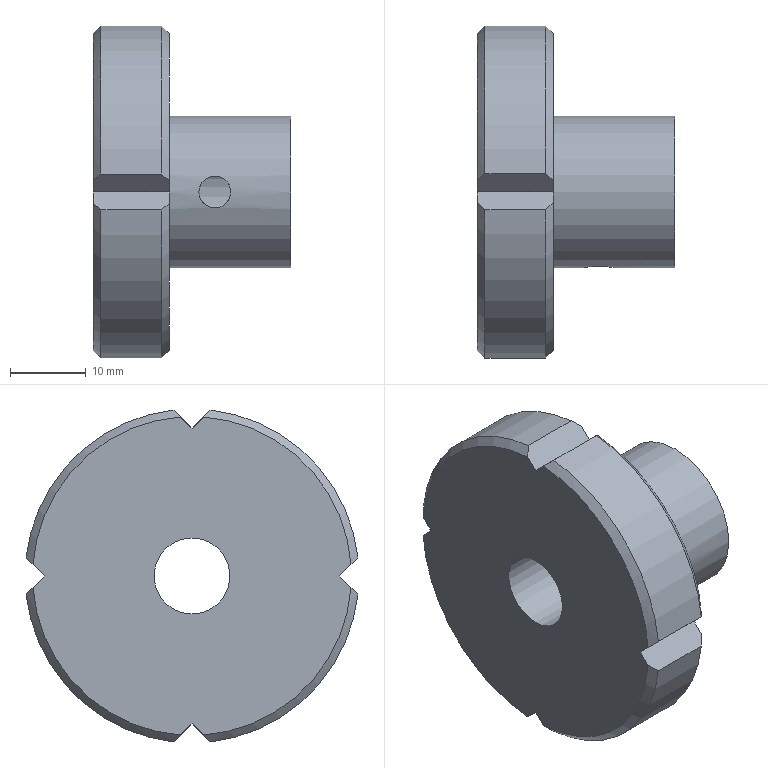Component | NX | 10_HANDLE | 1 solid | 26 faces | volume 17759 mm3 | plane 11 | cone 8 | cylinder 7 | commonest cylinder face diameters 44 x4 10 x1 20 x1 4.2 x1